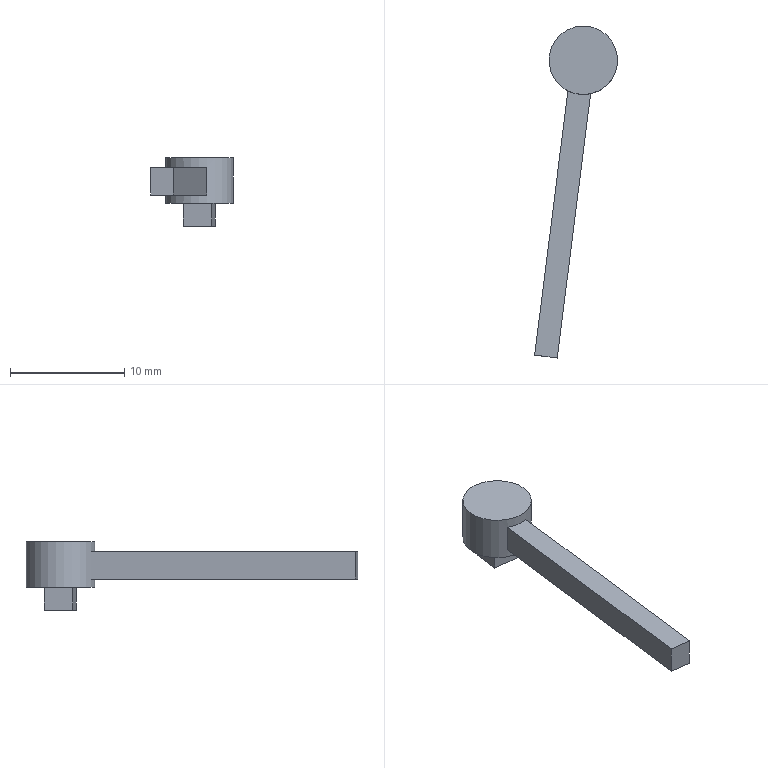Component | NX | HANDLE | 1 solid | 13 faces | box 7.27 x 29.03 x 6 mm | volume 237 mm3 | plane 12 | cylinder 1 | commonest cylinder face diameters 6 x1
STEP:
#1=CARTESIAN_POINT('',(0.,0.,0.));
#2=DIRECTION('',(0.,0.,1.));
#3=DIRECTION('',(1.,0.,0.));
#4=AXIS2_PLACEMENT_3D('',#1,#2,#3);
#5=CARTESIAN_POINT('',(33.486,50.648,24.212));
#6=VERTEX_POINT('',#5);
#7=CARTESIAN_POINT('',(30.51,51.025,24.212));
#8=DIRECTION('',(0.,0.,1.));
#9=DIRECTION('',(0.9921,-0.1255,0.));
#10=AXIS2_PLACEMENT_3D('',#7,#8,#9);
#11=CIRCLE('',#10,3.);
#12=CARTESIAN_POINT('',(30.51,51.025,24.212));
#13=DIRECTION('',(0.,0.,1.));
#14=DIRECTION('',(0.9921,-0.1255,0.));
#15=AXIS2_PLACEMENT_3D('',#12,#13,#14);
#16=CYLINDRICAL_SURFACE('',#15,3.);
#17=CARTESIAN_POINT('',(0.,0.));
#18=DIRECTION('',(1.,0.));
#19=VECTOR('',#18,1.);
#20=LINE('',#17,#19);
#21=(GEOMETRIC_REPRESENTATION_CONTEXT(2)PARAMETRIC_REPRESENTATION_CONTEXT()REPRESENTATION_CONTEXT('',''));
#22=DEFINITIONAL_REPRESENTATION('',(#20),#21);
#23=PCURVE('',#16,#22);
#24=CARTESIAN_POINT('',(30.51,51.025,24.212));
#25=DIRECTION('',(0.,0.,1.));
#26=DIRECTION('',(0.9921,-0.1255,0.));
#27=AXIS2_PLACEMENT_3D('',#24,#25,#26);
#28=PLANE('',#27);
#29=CARTESIAN_POINT('',(0.,0.));
#30=DIRECTION('',(1.,0.));
#31=AXIS2_PLACEMENT_2D('',#29,#30);
#32=CIRCLE('',#31,3.);
#33=(GEOMETRIC_REPRESENTATION_CONTEXT(2)PARAMETRIC_REPRESENTATION_CONTEXT()REPRESENTATION_CONTEXT('',''));
#34=DEFINITIONAL_REPRESENTATION('',(#32),#33);
#35=PCURVE('',#28,#34);
#36=SURFACE_CURVE('',#11,(#23,#35),.PCURVE_S1.);
#37=EDGE_CURVE('',#6,#6,#36,.T.);
#38=ORIENTED_EDGE('',*,*,#37,.T.);
#39=CARTESIAN_POINT('',(33.486,50.648,28.212));
#40=VERTEX_POINT('',#39);
#41=CARTESIAN_POINT('',(33.486,50.648,24.212));
#42=CARTESIAN_POINT('',(33.486,50.648,28.212));
#43=B_SPLINE_CURVE_WITH_KNOTS('',1,(#41,#42),.UNSPECIFIED.,.F.,.F.,(2,2),(0.,4.),.PIECEWISE_BEZIER_KNOTS.);
#44=CARTESIAN_POINT('',(6.283,0.));
#45=DIRECTION('',(0.,1.));
#46=VECTOR('',#45,1.);
#47=LINE('',#44,#46);
#48=(GEOMETRIC_REPRESENTATION_CONTEXT(2)PARAMETRIC_REPRESENTATION_CONTEXT()REPRESENTATION_CONTEXT('',''));
#49=DEFINITIONAL_REPRESENTATION('',(#47),#48);
#50=PCURVE('',#16,#49);
#51=CARTESIAN_POINT('',(0.,0.));
#52=DIRECTION('',(0.,1.));
#53=VECTOR('',#52,1.);
#54=LINE('',#51,#53);
#55=(GEOMETRIC_REPRESENTATION_CONTEXT(2)PARAMETRIC_REPRESENTATION_CONTEXT()REPRESENTATION_CONTEXT('',''));
#56=DEFINITIONAL_REPRESENTATION('',(#54),#55);
#57=PCURVE('',#16,#56);
#58=SEAM_CURVE('',#43,(#50,#57),.PCURVE_S1.);
#59=EDGE_CURVE('',#6,#40,#58,.T.);
#60=ORIENTED_EDGE('',*,*,#59,.T.);
#61=CARTESIAN_POINT('',(30.51,51.025,28.212));
#62=DIRECTION('',(0.,0.,1.));
#63=DIRECTION('',(0.9921,-0.1255,0.));
#64=AXIS2_PLACEMENT_3D('',#61,#62,#63);
#65=CIRCLE('',#64,3.);
#66=CARTESIAN_POINT('',(0.,4.));
#67=DIRECTION('',(1.,0.));
#68=VECTOR('',#67,1.);
#69=LINE('',#66,#68);
#70=(GEOMETRIC_REPRESENTATION_CONTEXT(2)PARAMETRIC_REPRESENTATION_CONTEXT()REPRESENTATION_CONTEXT('',''));
#71=DEFINITIONAL_REPRESENTATION('',(#69),#70);
#72=PCURVE('',#16,#71);
#73=CARTESIAN_POINT('',(30.51,51.025,28.212));
#74=DIRECTION('',(0.,0.,1.));
#75=DIRECTION('',(0.9921,-0.1255,0.));
#76=AXIS2_PLACEMENT_3D('',#73,#74,#75);
#77=PLANE('',#76);
#78=CARTESIAN_POINT('',(0.,0.));
#79=DIRECTION('',(1.,0.));
#80=AXIS2_PLACEMENT_2D('',#78,#79);
#81=CIRCLE('',#80,3.);
#82=(GEOMETRIC_REPRESENTATION_CONTEXT(2)PARAMETRIC_REPRESENTATION_CONTEXT()REPRESENTATION_CONTEXT('',''));
#83=DEFINITIONAL_REPRESENTATION('',(#81),#82);
#84=PCURVE('',#77,#83);
#85=SURFACE_CURVE('',#65,(#72,#84),.PCURVE_S1.);
#86=EDGE_CURVE('',#40,#40,#85,.T.);
#87=ORIENTED_EDGE('',*,*,#86,.F.);
#88=ORIENTED_EDGE('',*,*,#59,.F.);
#89=EDGE_LOOP('',(#38,#60,#87,#88));
#90=FACE_BOUND('',#89,.T.);
#91=CARTESIAN_POINT('',(29.163,48.344,24.948));
#92=VERTEX_POINT('',#91);
#93=CARTESIAN_POINT('',(31.147,48.093,24.948));
#94=VERTEX_POINT('',#93);
#95=CARTESIAN_POINT('',(30.51,51.025,24.948));
#96=DIRECTION('',(0.,0.,1.));
#97=DIRECTION('',(-0.9921,0.1255,0.));
#98=AXIS2_PLACEMENT_3D('',#95,#96,#97);
#99=CIRCLE('',#98,3.);
#100=CARTESIAN_POINT('',(3.142,0.7363));
#101=DIRECTION('',(1.,0.));
#102=VECTOR('',#101,1.);
#103=LINE('',#100,#102);
#104=(GEOMETRIC_REPRESENTATION_CONTEXT(2)PARAMETRIC_REPRESENTATION_CONTEXT()REPRESENTATION_CONTEXT('',''));
#105=DEFINITIONAL_REPRESENTATION('',(#103),#104);
#106=PCURVE('',#16,#105);
#107=CARTESIAN_POINT('',(26.242,25.242,24.948));
#108=DIRECTION('',(0.,0.,-1.));
#109=DIRECTION('',(-0.9921,0.1255,0.));
#110=AXIS2_PLACEMENT_3D('',#107,#108,#109);
#111=PLANE('',#110);
#112=CARTESIAN_POINT('',(2.,26.115));
#113=CARTESIAN_POINT('',(2.,20.919));
#114=CARTESIAN_POINT('',(-2.5,23.517));
#115=CARTESIAN_POINT('',(-7.,26.115));
#116=CARTESIAN_POINT('',(-2.5,28.713));
#117=CARTESIAN_POINT('',(2.,31.311));
#118=CARTESIAN_POINT('',(2.,26.115));
#119=(BOUNDED_CURVE()B_SPLINE_CURVE(2,(#112,#113,#114,#115,#116,#117,#118),.UNSPECIFIED.,.T.,.F.)B_SPLINE_CURVE_WITH_KNOTS((1,2,2,2,2,1),(-2.094,0.,2.094,4.189,6.283,8.378),.UNSPECIFIED.)CURVE()GEOMETRIC_REPRESENTATION_ITEM()RATIONAL_B_SPLINE_CURVE((1.,0.5,1.,0.5,1.,0.5,1.))REPRESENTATION_ITEM(''));
#120=(GEOMETRIC_REPRESENTATION_CONTEXT(2)PARAMETRIC_REPRESENTATION_CONTEXT()REPRESENTATION_CONTEXT('',''));
#121=DEFINITIONAL_REPRESENTATION('',(#119),#120);
#122=PCURVE('',#111,#121);
#123=SURFACE_CURVE('',#99,(#106,#122),.PCURVE_S1.);
#124=EDGE_CURVE('',#92,#94,#123,.T.);
#125=ORIENTED_EDGE('',*,*,#124,.F.);
#126=CARTESIAN_POINT('',(29.163,48.344,27.342));
#127=VERTEX_POINT('',#126);
#128=CARTESIAN_POINT('',(29.163,48.344,24.212));
#129=DIRECTION('',(0.,0.,1.));
#130=VECTOR('',#129,1.);
#131=LINE('',#128,#130);
#132=CARTESIAN_POINT('',(4.373,0.));
#133=DIRECTION('',(0.,1.));
#134=VECTOR('',#133,1.);
#135=LINE('',#132,#134);
#136=(GEOMETRIC_REPRESENTATION_CONTEXT(2)PARAMETRIC_REPRESENTATION_CONTEXT()REPRESENTATION_CONTEXT('',''));
#137=DEFINITIONAL_REPRESENTATION('',(#135),#136);
#138=PCURVE('',#16,#137);
#139=CARTESIAN_POINT('',(29.518,51.15,24.212));
#140=DIRECTION('',(0.9921,-0.1255,0.));
#141=DIRECTION('',(0.,0.,-1.));
#142=AXIS2_PLACEMENT_3D('',#139,#140,#141);
#143=PLANE('',#142);
#144=CARTESIAN_POINT('',(0.,-2.828));
#145=DIRECTION('',(-1.,0.));
#146=VECTOR('',#145,1.);
#147=LINE('',#144,#146);
#148=(GEOMETRIC_REPRESENTATION_CONTEXT(2)PARAMETRIC_REPRESENTATION_CONTEXT()REPRESENTATION_CONTEXT('',''));
#149=DEFINITIONAL_REPRESENTATION('',(#147),#148);
#150=PCURVE('',#143,#149);
#151=SURFACE_CURVE('',#131,(#138,#150),.PCURVE_S1.);
#152=EDGE_CURVE('',#92,#127,#151,.T.);
#153=ORIENTED_EDGE('',*,*,#152,.T.);
#154=CARTESIAN_POINT('',(31.147,48.093,27.342));
#155=VERTEX_POINT('',#154);
#156=CARTESIAN_POINT('',(30.51,51.025,27.342));
#157=DIRECTION('',(0.,0.,-1.));
#158=DIRECTION('',(-0.1255,-0.9921,-0.));
#159=AXIS2_PLACEMENT_3D('',#156,#157,#158);
#160=CIRCLE('',#159,3.);
#161=CARTESIAN_POINT('',(10.996,3.13));
#162=DIRECTION('',(-1.,0.));
#163=VECTOR('',#162,1.);
#164=LINE('',#161,#163);
#165=(GEOMETRIC_REPRESENTATION_CONTEXT(2)PARAMETRIC_REPRESENTATION_CONTEXT()REPRESENTATION_CONTEXT('',''));
#166=DEFINITIONAL_REPRESENTATION('',(#164),#165);
#167=PCURVE('',#16,#166);
#168=CARTESIAN_POINT('',(29.417,50.356,27.342));
#169=DIRECTION('',(-0.,-0.,1.));
#170=DIRECTION('',(-0.1255,-0.9921,-0.));
#171=AXIS2_PLACEMENT_3D('',#168,#169,#170);
#172=PLANE('',#171);
#173=CARTESIAN_POINT('',(2.2,1.));
#174=CARTESIAN_POINT('',(2.2,-4.196));
#175=CARTESIAN_POINT('',(-2.3,-1.598));
#176=CARTESIAN_POINT('',(-6.8,1.));
#177=CARTESIAN_POINT('',(-2.3,3.598));
#178=CARTESIAN_POINT('',(2.2,6.196));
#179=CARTESIAN_POINT('',(2.2,1.));
#180=(BOUNDED_CURVE()B_SPLINE_CURVE(2,(#173,#174,#175,#176,#177,#178,#179),.UNSPECIFIED.,.T.,.F.)B_SPLINE_CURVE_WITH_KNOTS((1,2,2,2,2,1),(-2.094,0.,2.094,4.189,6.283,8.378),.UNSPECIFIED.)CURVE()GEOMETRIC_REPRESENTATION_ITEM()RATIONAL_B_SPLINE_CURVE((1.,0.5,1.,0.5,1.,0.5,1.))REPRESENTATION_ITEM(''));
#181=(GEOMETRIC_REPRESENTATION_CONTEXT(2)PARAMETRIC_REPRESENTATION_CONTEXT()REPRESENTATION_CONTEXT('',''));
#182=DEFINITIONAL_REPRESENTATION('',(#180),#181);
#183=PCURVE('',#172,#182);
#184=SURFACE_CURVE('',#160,(#167,#183),.PCURVE_S1.);
#185=EDGE_CURVE('',#155,#127,#184,.T.);
#186=ORIENTED_EDGE('',*,*,#185,.F.);
#187=CARTESIAN_POINT('',(31.147,48.093,24.212));
#188=DIRECTION('',(0.,0.,1.));
#189=VECTOR('',#188,1.);
#190=LINE('',#187,#189);
#191=CARTESIAN_POINT('',(5.052,0.));
#192=DIRECTION('',(0.,1.));
#193=VECTOR('',#192,1.);
#194=LINE('',#191,#193);
#195=(GEOMETRIC_REPRESENTATION_CONTEXT(2)PARAMETRIC_REPRESENTATION_CONTEXT()REPRESENTATION_CONTEXT('',''));
#196=DEFINITIONAL_REPRESENTATION('',(#194),#195);
#197=PCURVE('',#16,#196);
#198=CARTESIAN_POINT('',(31.502,50.899,24.212));
#199=DIRECTION('',(0.9921,-0.1255,0.));
#200=DIRECTION('',(0.,0.,-1.));
#201=AXIS2_PLACEMENT_3D('',#198,#199,#200);
#202=PLANE('',#201);
#203=CARTESIAN_POINT('',(0.,-2.828));
#204=DIRECTION('',(-1.,0.));
#205=VECTOR('',#204,1.);
#206=LINE('',#203,#205);
#207=(GEOMETRIC_REPRESENTATION_CONTEXT(2)PARAMETRIC_REPRESENTATION_CONTEXT()REPRESENTATION_CONTEXT('',''));
#208=DEFINITIONAL_REPRESENTATION('',(#206),#207);
#209=PCURVE('',#202,#208);
#210=SURFACE_CURVE('',#190,(#197,#209),.PCURVE_S1.);
#211=EDGE_CURVE('',#94,#155,#210,.T.);
#212=ORIENTED_EDGE('',*,*,#211,.F.);
#213=EDGE_LOOP('',(#125,#153,#186,#212));
#214=FACE_BOUND('',#213,.T.);
#215=ADVANCED_FACE('',(#90,#214),#16,.T.);
#216=ORIENTED_EDGE('',*,*,#37,.F.);
#217=EDGE_LOOP('',(#216));
#218=FACE_BOUND('',#217,.T.);
#219=CARTESIAN_POINT('',(29.113,49.941,24.212));
#220=VERTEX_POINT('',#219);
#221=CARTESIAN_POINT('',(29.427,52.422,24.212));
#222=VERTEX_POINT('',#221);
#223=CARTESIAN_POINT('',(29.113,49.941,24.212));
#224=DIRECTION('',(0.1255,0.9921,0.));
#225=VECTOR('',#224,1.);
#226=LINE('',#223,#225);
#227=CARTESIAN_POINT('',(-1.25,-1.25));
#228=DIRECTION('',(0.,1.));
#229=VECTOR('',#228,1.);
#230=LINE('',#227,#229);
#231=(GEOMETRIC_REPRESENTATION_CONTEXT(2)PARAMETRIC_REPRESENTATION_CONTEXT()REPRESENTATION_CONTEXT('',''));
#232=DEFINITIONAL_REPRESENTATION('',(#230),#231);
#233=PCURVE('',#28,#232);
#234=CARTESIAN_POINT('',(29.427,52.422,22.212));
#235=DIRECTION('',(-0.9921,0.1255,0.));
#236=DIRECTION('',(0.,0.,1.));
#237=AXIS2_PLACEMENT_3D('',#234,#235,#236);
#238=PLANE('',#237);
#239=CARTESIAN_POINT('',(2.,-2.5));
#240=DIRECTION('',(0.,1.));
#241=VECTOR('',#240,1.);
#242=LINE('',#239,#241);
#243=(GEOMETRIC_REPRESENTATION_CONTEXT(2)PARAMETRIC_REPRESENTATION_CONTEXT()REPRESENTATION_CONTEXT('',''));
#244=DEFINITIONAL_REPRESENTATION('',(#242),#243);
#245=PCURVE('',#238,#244);
#246=SURFACE_CURVE('',#226,(#233,#245),.PCURVE_S1.);
#247=EDGE_CURVE('',#220,#222,#246,.T.);
#248=ORIENTED_EDGE('',*,*,#247,.F.);
#249=CARTESIAN_POINT('',(31.593,49.628,24.212));
#250=VERTEX_POINT('',#249);
#251=CARTESIAN_POINT('',(31.593,49.628,24.212));
#252=DIRECTION('',(-0.9921,0.1255,0.));
#253=VECTOR('',#252,1.);
#254=LINE('',#251,#253);
#255=CARTESIAN_POINT('',(1.25,-1.25));
#256=DIRECTION('',(-1.,0.));
#257=VECTOR('',#256,1.);
#258=LINE('',#255,#257);
#259=(GEOMETRIC_REPRESENTATION_CONTEXT(2)PARAMETRIC_REPRESENTATION_CONTEXT()REPRESENTATION_CONTEXT('',''));
#260=DEFINITIONAL_REPRESENTATION('',(#258),#259);
#261=PCURVE('',#28,#260);
#262=CARTESIAN_POINT('',(29.113,49.941,22.212));
#263=DIRECTION('',(-0.1255,-0.9921,0.));
#264=DIRECTION('',(0.9921,-0.1255,0.));
#265=AXIS2_PLACEMENT_3D('',#262,#263,#264);
#266=PLANE('',#265);
#267=CARTESIAN_POINT('',(2.5,2.));
#268=DIRECTION('',(-1.,0.));
#269=VECTOR('',#268,1.);
#270=LINE('',#267,#269);
#271=(GEOMETRIC_REPRESENTATION_CONTEXT(2)PARAMETRIC_REPRESENTATION_CONTEXT()REPRESENTATION_CONTEXT('',''));
#272=DEFINITIONAL_REPRESENTATION('',(#270),#271);
#273=PCURVE('',#266,#272);
#274=SURFACE_CURVE('',#254,(#261,#273),.PCURVE_S1.);
#275=EDGE_CURVE('',#250,#220,#274,.T.);
#276=ORIENTED_EDGE('',*,*,#275,.F.);
#277=CARTESIAN_POINT('',(31.907,52.108,24.212));
#278=VERTEX_POINT('',#277);
#279=CARTESIAN_POINT('',(31.907,52.108,24.212));
#280=DIRECTION('',(-0.1255,-0.9921,0.));
#281=VECTOR('',#280,1.);
#282=LINE('',#279,#281);
#283=CARTESIAN_POINT('',(1.25,1.25));
#284=DIRECTION('',(0.,-1.));
#285=VECTOR('',#284,1.);
#286=LINE('',#283,#285);
#287=(GEOMETRIC_REPRESENTATION_CONTEXT(2)PARAMETRIC_REPRESENTATION_CONTEXT()REPRESENTATION_CONTEXT('',''));
#288=DEFINITIONAL_REPRESENTATION('',(#286),#287);
#289=PCURVE('',#28,#288);
#290=CARTESIAN_POINT('',(31.593,49.628,22.212));
#291=DIRECTION('',(0.9921,-0.1255,0.));
#292=DIRECTION('',(0.1255,0.9921,0.));
#293=AXIS2_PLACEMENT_3D('',#290,#291,#292);
#294=PLANE('',#293);
#295=CARTESIAN_POINT('',(2.5,2.));
#296=DIRECTION('',(-1.,0.));
#297=VECTOR('',#296,1.);
#298=LINE('',#295,#297);
#299=(GEOMETRIC_REPRESENTATION_CONTEXT(2)PARAMETRIC_REPRESENTATION_CONTEXT()REPRESENTATION_CONTEXT('',''));
#300=DEFINITIONAL_REPRESENTATION('',(#298),#299);
#301=PCURVE('',#294,#300);
#302=SURFACE_CURVE('',#282,(#289,#301),.PCURVE_S1.);
#303=EDGE_CURVE('',#278,#250,#302,.T.);
#304=ORIENTED_EDGE('',*,*,#303,.F.);
#305=CARTESIAN_POINT('',(29.427,52.422,24.212));
#306=DIRECTION('',(0.9921,-0.1255,0.));
#307=VECTOR('',#306,1.);
#308=LINE('',#305,#307);
#309=CARTESIAN_POINT('',(-1.25,1.25));
#310=DIRECTION('',(1.,0.));
#311=VECTOR('',#310,1.);
#312=LINE('',#309,#311);
#313=(GEOMETRIC_REPRESENTATION_CONTEXT(2)PARAMETRIC_REPRESENTATION_CONTEXT()REPRESENTATION_CONTEXT('',''));
#314=DEFINITIONAL_REPRESENTATION('',(#312),#313);
#315=PCURVE('',#28,#314);
#316=CARTESIAN_POINT('',(31.907,52.108,22.212));
#317=DIRECTION('',(0.1255,0.9921,0.));
#318=DIRECTION('',(-0.9921,0.1255,0.));
#319=AXIS2_PLACEMENT_3D('',#316,#317,#318);
#320=PLANE('',#319);
#321=CARTESIAN_POINT('',(2.5,2.));
#322=DIRECTION('',(-1.,0.));
#323=VECTOR('',#322,1.);
#324=LINE('',#321,#323);
#325=(GEOMETRIC_REPRESENTATION_CONTEXT(2)PARAMETRIC_REPRESENTATION_CONTEXT()REPRESENTATION_CONTEXT('',''));
#326=DEFINITIONAL_REPRESENTATION('',(#324),#325);
#327=PCURVE('',#320,#326);
#328=SURFACE_CURVE('',#308,(#315,#327),.PCURVE_S1.);
#329=EDGE_CURVE('',#222,#278,#328,.T.);
#330=ORIENTED_EDGE('',*,*,#329,.F.);
#331=EDGE_LOOP('',(#248,#276,#304,#330));
#332=FACE_BOUND('',#331,.T.);
#333=ADVANCED_FACE('',(#218,#332),#28,.F.);
#334=ORIENTED_EDGE('',*,*,#86,.T.);
#335=EDGE_LOOP('',(#334));
#336=FACE_BOUND('',#335,.T.);
#337=ADVANCED_FACE('',(#336),#77,.T.);
#338=CARTESIAN_POINT('',(29.427,52.422,22.212));
#339=VERTEX_POINT('',#338);
#340=CARTESIAN_POINT('',(29.113,49.941,22.212));
#341=VERTEX_POINT('',#340);
#342=CARTESIAN_POINT('',(29.427,52.422,22.212));
#343=DIRECTION('',(-0.1255,-0.9921,0.));
#344=VECTOR('',#343,1.);
#345=LINE('',#342,#344);
#346=CARTESIAN_POINT('',(30.51,51.025,22.212));
#347=DIRECTION('',(0.,0.,1.));
#348=DIRECTION('',(0.9921,-0.1255,0.));
#349=AXIS2_PLACEMENT_3D('',#346,#347,#348);
#350=PLANE('',#349);
#351=CARTESIAN_POINT('',(-1.25,1.25));
#352=DIRECTION('',(0.,-1.));
#353=VECTOR('',#352,1.);
#354=LINE('',#351,#353);
#355=(GEOMETRIC_REPRESENTATION_CONTEXT(2)PARAMETRIC_REPRESENTATION_CONTEXT()REPRESENTATION_CONTEXT('',''));
#356=DEFINITIONAL_REPRESENTATION('',(#354),#355);
#357=PCURVE('',#350,#356);
#358=CARTESIAN_POINT('',(0.,0.));
#359=DIRECTION('',(0.,-1.));
#360=VECTOR('',#359,1.);
#361=LINE('',#358,#360);
#362=(GEOMETRIC_REPRESENTATION_CONTEXT(2)PARAMETRIC_REPRESENTATION_CONTEXT()REPRESENTATION_CONTEXT('',''));
#363=DEFINITIONAL_REPRESENTATION('',(#361),#362);
#364=PCURVE('',#238,#363);
#365=SURFACE_CURVE('',#345,(#357,#364),.PCURVE_S1.);
#366=EDGE_CURVE('',#339,#341,#365,.T.);
#367=ORIENTED_EDGE('',*,*,#366,.F.);
#368=CARTESIAN_POINT('',(31.907,52.108,22.212));
#369=VERTEX_POINT('',#368);
#370=CARTESIAN_POINT('',(31.907,52.108,22.212));
#371=DIRECTION('',(-0.9921,0.1255,0.));
#372=VECTOR('',#371,1.);
#373=LINE('',#370,#372);
#374=CARTESIAN_POINT('',(1.25,1.25));
#375=DIRECTION('',(-1.,0.));
#376=VECTOR('',#375,1.);
#377=LINE('',#374,#376);
#378=(GEOMETRIC_REPRESENTATION_CONTEXT(2)PARAMETRIC_REPRESENTATION_CONTEXT()REPRESENTATION_CONTEXT('',''));
#379=DEFINITIONAL_REPRESENTATION('',(#377),#378);
#380=PCURVE('',#350,#379);
#381=CARTESIAN_POINT('',(0.,0.));
#382=DIRECTION('',(1.,0.));
#383=VECTOR('',#382,1.);
#384=LINE('',#381,#383);
#385=(GEOMETRIC_REPRESENTATION_CONTEXT(2)PARAMETRIC_REPRESENTATION_CONTEXT()REPRESENTATION_CONTEXT('',''));
#386=DEFINITIONAL_REPRESENTATION('',(#384),#385);
#387=PCURVE('',#320,#386);
#388=SURFACE_CURVE('',#373,(#380,#387),.PCURVE_S1.);
#389=EDGE_CURVE('',#369,#339,#388,.T.);
#390=ORIENTED_EDGE('',*,*,#389,.F.);
#391=CARTESIAN_POINT('',(31.593,49.628,22.212));
#392=VERTEX_POINT('',#391);
#393=CARTESIAN_POINT('',(31.593,49.628,22.212));
#394=DIRECTION('',(0.1255,0.9921,0.));
#395=VECTOR('',#394,1.);
#396=LINE('',#393,#395);
#397=CARTESIAN_POINT('',(1.25,-1.25));
#398=DIRECTION('',(0.,1.));
#399=VECTOR('',#398,1.);
#400=LINE('',#397,#399);
#401=(GEOMETRIC_REPRESENTATION_CONTEXT(2)PARAMETRIC_REPRESENTATION_CONTEXT()REPRESENTATION_CONTEXT('',''));
#402=DEFINITIONAL_REPRESENTATION('',(#400),#401);
#403=PCURVE('',#350,#402);
#404=CARTESIAN_POINT('',(0.,0.));
#405=DIRECTION('',(1.,0.));
#406=VECTOR('',#405,1.);
#407=LINE('',#404,#406);
#408=(GEOMETRIC_REPRESENTATION_CONTEXT(2)PARAMETRIC_REPRESENTATION_CONTEXT()REPRESENTATION_CONTEXT('',''));
#409=DEFINITIONAL_REPRESENTATION('',(#407),#408);
#410=PCURVE('',#294,#409);
#411=SURFACE_CURVE('',#396,(#403,#410),.PCURVE_S1.);
#412=EDGE_CURVE('',#392,#369,#411,.T.);
#413=ORIENTED_EDGE('',*,*,#412,.F.);
#414=CARTESIAN_POINT('',(29.113,49.941,22.212));
#415=DIRECTION('',(0.9921,-0.1255,0.));
#416=VECTOR('',#415,1.);
#417=LINE('',#414,#416);
#418=CARTESIAN_POINT('',(-1.25,-1.25));
#419=DIRECTION('',(1.,0.));
#420=VECTOR('',#419,1.);
#421=LINE('',#418,#420);
#422=(GEOMETRIC_REPRESENTATION_CONTEXT(2)PARAMETRIC_REPRESENTATION_CONTEXT()REPRESENTATION_CONTEXT('',''));
#423=DEFINITIONAL_REPRESENTATION('',(#421),#422);
#424=PCURVE('',#350,#423);
#425=CARTESIAN_POINT('',(0.,0.));
#426=DIRECTION('',(1.,0.));
#427=VECTOR('',#426,1.);
#428=LINE('',#425,#427);
#429=(GEOMETRIC_REPRESENTATION_CONTEXT(2)PARAMETRIC_REPRESENTATION_CONTEXT()REPRESENTATION_CONTEXT('',''));
#430=DEFINITIONAL_REPRESENTATION('',(#428),#429);
#431=PCURVE('',#266,#430);
#432=SURFACE_CURVE('',#417,(#424,#431),.PCURVE_S1.);
#433=EDGE_CURVE('',#341,#392,#432,.T.);
#434=ORIENTED_EDGE('',*,*,#433,.F.);
#435=EDGE_LOOP('',(#367,#390,#413,#434));
#436=FACE_BOUND('',#435,.T.);
#437=ADVANCED_FACE('',(#436),#350,.F.);
#438=ORIENTED_EDGE('',*,*,#329,.T.);
#439=CARTESIAN_POINT('',(31.907,52.108,22.212));
#440=DIRECTION('',(0.,0.,1.));
#441=VECTOR('',#440,1.);
#442=LINE('',#439,#441);
#443=CARTESIAN_POINT('',(0.,0.));
#444=DIRECTION('',(0.,1.));
#445=VECTOR('',#444,1.);
#446=LINE('',#443,#445);
#447=(GEOMETRIC_REPRESENTATION_CONTEXT(2)PARAMETRIC_REPRESENTATION_CONTEXT()REPRESENTATION_CONTEXT('',''));
#448=DEFINITIONAL_REPRESENTATION('',(#446),#447);
#449=PCURVE('',#320,#448);
#450=CARTESIAN_POINT('',(2.5,0.));
#451=DIRECTION('',(0.,1.));
#452=VECTOR('',#451,1.);
#453=LINE('',#450,#452);
#454=(GEOMETRIC_REPRESENTATION_CONTEXT(2)PARAMETRIC_REPRESENTATION_CONTEXT()REPRESENTATION_CONTEXT('',''));
#455=DEFINITIONAL_REPRESENTATION('',(#453),#454);
#456=PCURVE('',#294,#455);
#457=SURFACE_CURVE('',#442,(#449,#456),.PCURVE_S1.);
#458=EDGE_CURVE('',#369,#278,#457,.T.);
#459=ORIENTED_EDGE('',*,*,#458,.F.);
#460=ORIENTED_EDGE('',*,*,#389,.T.);
#461=CARTESIAN_POINT('',(29.427,52.422,22.212));
#462=DIRECTION('',(0.,0.,1.));
#463=VECTOR('',#462,1.);
#464=LINE('',#461,#463);
#465=CARTESIAN_POINT('',(2.5,0.));
#466=DIRECTION('',(0.,1.));
#467=VECTOR('',#466,1.);
#468=LINE('',#465,#467);
#469=(GEOMETRIC_REPRESENTATION_CONTEXT(2)PARAMETRIC_REPRESENTATION_CONTEXT()REPRESENTATION_CONTEXT('',''));
#470=DEFINITIONAL_REPRESENTATION('',(#468),#469);
#471=PCURVE('',#320,#470);
#472=CARTESIAN_POINT('',(0.,0.));
#473=DIRECTION('',(1.,0.));
#474=VECTOR('',#473,1.);
#475=LINE('',#472,#474);
#476=(GEOMETRIC_REPRESENTATION_CONTEXT(2)PARAMETRIC_REPRESENTATION_CONTEXT()REPRESENTATION_CONTEXT('',''));
#477=DEFINITIONAL_REPRESENTATION('',(#475),#476);
#478=PCURVE('',#238,#477);
#479=SURFACE_CURVE('',#464,(#471,#478),.PCURVE_S1.);
#480=EDGE_CURVE('',#339,#222,#479,.T.);
#481=ORIENTED_EDGE('',*,*,#480,.T.);
#482=EDGE_LOOP('',(#438,#459,#460,#481));
#483=FACE_BOUND('',#482,.T.);
#484=ADVANCED_FACE('',(#483),#320,.T.);
#485=ORIENTED_EDGE('',*,*,#303,.T.);
#486=CARTESIAN_POINT('',(31.593,49.628,22.212));
#487=DIRECTION('',(0.,0.,1.));
#488=VECTOR('',#487,1.);
#489=LINE('',#486,#488);
#490=CARTESIAN_POINT('',(0.,0.));
#491=DIRECTION('',(0.,1.));
#492=VECTOR('',#491,1.);
#493=LINE('',#490,#492);
#494=(GEOMETRIC_REPRESENTATION_CONTEXT(2)PARAMETRIC_REPRESENTATION_CONTEXT()REPRESENTATION_CONTEXT('',''));
#495=DEFINITIONAL_REPRESENTATION('',(#493),#494);
#496=PCURVE('',#294,#495);
#497=CARTESIAN_POINT('',(2.5,0.));
#498=DIRECTION('',(0.,1.));
#499=VECTOR('',#498,1.);
#500=LINE('',#497,#499);
#501=(GEOMETRIC_REPRESENTATION_CONTEXT(2)PARAMETRIC_REPRESENTATION_CONTEXT()REPRESENTATION_CONTEXT('',''));
#502=DEFINITIONAL_REPRESENTATION('',(#500),#501);
#503=PCURVE('',#266,#502);
#504=SURFACE_CURVE('',#489,(#496,#503),.PCURVE_S1.);
#505=EDGE_CURVE('',#392,#250,#504,.T.);
#506=ORIENTED_EDGE('',*,*,#505,.F.);
#507=ORIENTED_EDGE('',*,*,#412,.T.);
#508=ORIENTED_EDGE('',*,*,#458,.T.);
#509=EDGE_LOOP('',(#485,#506,#507,#508));
#510=FACE_BOUND('',#509,.T.);
#511=ADVANCED_FACE('',(#510),#294,.T.);
#512=ORIENTED_EDGE('',*,*,#275,.T.);
#513=CARTESIAN_POINT('',(29.113,49.941,22.212));
#514=DIRECTION('',(0.,0.,1.));
#515=VECTOR('',#514,1.);
#516=LINE('',#513,#515);
#517=CARTESIAN_POINT('',(0.,0.));
#518=DIRECTION('',(0.,1.));
#519=VECTOR('',#518,1.);
#520=LINE('',#517,#519);
#521=(GEOMETRIC_REPRESENTATION_CONTEXT(2)PARAMETRIC_REPRESENTATION_CONTEXT()REPRESENTATION_CONTEXT('',''));
#522=DEFINITIONAL_REPRESENTATION('',(#520),#521);
#523=PCURVE('',#266,#522);
#524=CARTESIAN_POINT('',(0.,-2.5));
#525=DIRECTION('',(1.,0.));
#526=VECTOR('',#525,1.);
#527=LINE('',#524,#526);
#528=(GEOMETRIC_REPRESENTATION_CONTEXT(2)PARAMETRIC_REPRESENTATION_CONTEXT()REPRESENTATION_CONTEXT('',''));
#529=DEFINITIONAL_REPRESENTATION('',(#527),#528);
#530=PCURVE('',#238,#529);
#531=SURFACE_CURVE('',#516,(#523,#530),.PCURVE_S1.);
#532=EDGE_CURVE('',#341,#220,#531,.T.);
#533=ORIENTED_EDGE('',*,*,#532,.F.);
#534=ORIENTED_EDGE('',*,*,#433,.T.);
#535=ORIENTED_EDGE('',*,*,#505,.T.);
#536=EDGE_LOOP('',(#512,#533,#534,#535));
#537=FACE_BOUND('',#536,.T.);
#538=ADVANCED_FACE('',(#537),#266,.T.);
#539=ORIENTED_EDGE('',*,*,#247,.T.);
#540=ORIENTED_EDGE('',*,*,#480,.F.);
#541=ORIENTED_EDGE('',*,*,#366,.T.);
#542=ORIENTED_EDGE('',*,*,#532,.T.);
#543=EDGE_LOOP('',(#539,#540,#541,#542));
#544=FACE_BOUND('',#543,.T.);
#545=ADVANCED_FACE('',(#544),#238,.T.);
#546=CARTESIAN_POINT('',(28.226,24.991,27.342));
#547=VERTEX_POINT('',#546);
#548=CARTESIAN_POINT('',(28.226,24.991,24.948));
#549=VERTEX_POINT('',#548);
#550=CARTESIAN_POINT('',(28.226,24.991,27.342));
#551=DIRECTION('',(0.,0.,-1.));
#552=VECTOR('',#551,1.);
#553=LINE('',#550,#552);
#554=CARTESIAN_POINT('',(26.242,25.242,27.342));
#555=DIRECTION('',(-0.1255,-0.9921,0.));
#556=DIRECTION('',(0.,0.,-1.));
#557=AXIS2_PLACEMENT_3D('',#554,#555,#556);
#558=PLANE('',#557);
#559=CARTESIAN_POINT('',(0.,2.));
#560=DIRECTION('',(1.,0.));
#561=VECTOR('',#560,1.);
#562=LINE('',#559,#561);
#563=(GEOMETRIC_REPRESENTATION_CONTEXT(2)PARAMETRIC_REPRESENTATION_CONTEXT()REPRESENTATION_CONTEXT('',''));
#564=DEFINITIONAL_REPRESENTATION('',(#562),#563);
#565=PCURVE('',#558,#564);
#566=CARTESIAN_POINT('',(-3.13,-26.115));
#567=DIRECTION('',(1.,0.));
#568=VECTOR('',#567,1.);
#569=LINE('',#566,#568);
#570=(GEOMETRIC_REPRESENTATION_CONTEXT(2)PARAMETRIC_REPRESENTATION_CONTEXT()REPRESENTATION_CONTEXT('',''));
#571=DEFINITIONAL_REPRESENTATION('',(#569),#570);
#572=PCURVE('',#202,#571);
#573=SURFACE_CURVE('',#553,(#565,#572),.PCURVE_S1.);
#574=EDGE_CURVE('',#547,#549,#573,.T.);
#575=ORIENTED_EDGE('',*,*,#574,.F.);
#576=CARTESIAN_POINT('',(26.242,25.242,27.342));
#577=VERTEX_POINT('',#576);
#578=CARTESIAN_POINT('',(26.242,25.242,27.342));
#579=DIRECTION('',(0.9921,-0.1255,0.));
#580=VECTOR('',#579,1.);
#581=LINE('',#578,#580);
#582=CARTESIAN_POINT('',(0.,0.));
#583=DIRECTION('',(0.,1.));
#584=VECTOR('',#583,1.);
#585=LINE('',#582,#584);
#586=(GEOMETRIC_REPRESENTATION_CONTEXT(2)PARAMETRIC_REPRESENTATION_CONTEXT()REPRESENTATION_CONTEXT('',''));
#587=DEFINITIONAL_REPRESENTATION('',(#585),#586);
#588=PCURVE('',#558,#587);
#589=CARTESIAN_POINT('',(25.315,0.));
#590=DIRECTION('',(0.,1.));
#591=VECTOR('',#590,1.);
#592=LINE('',#589,#591);
#593=(GEOMETRIC_REPRESENTATION_CONTEXT(2)PARAMETRIC_REPRESENTATION_CONTEXT()REPRESENTATION_CONTEXT('',''));
#594=DEFINITIONAL_REPRESENTATION('',(#592),#593);
#595=PCURVE('',#172,#594);
#596=SURFACE_CURVE('',#581,(#588,#595),.PCURVE_S1.);
#597=EDGE_CURVE('',#577,#547,#596,.T.);
#598=ORIENTED_EDGE('',*,*,#597,.F.);
#599=CARTESIAN_POINT('',(26.242,25.242,24.948));
#600=VERTEX_POINT('',#599);
#601=CARTESIAN_POINT('',(26.242,25.242,27.342));
#602=DIRECTION('',(0.,0.,-1.));
#603=VECTOR('',#602,1.);
#604=LINE('',#601,#603);
#605=CARTESIAN_POINT('',(0.,0.));
#606=DIRECTION('',(1.,0.));
#607=VECTOR('',#606,1.);
#608=LINE('',#605,#607);
#609=(GEOMETRIC_REPRESENTATION_CONTEXT(2)PARAMETRIC_REPRESENTATION_CONTEXT()REPRESENTATION_CONTEXT('',''));
#610=DEFINITIONAL_REPRESENTATION('',(#608),#609);
#611=PCURVE('',#558,#610);
#612=CARTESIAN_POINT('',(-3.13,-26.115));
#613=DIRECTION('',(1.,0.));
#614=VECTOR('',#613,1.);
#615=LINE('',#612,#614);
#616=(GEOMETRIC_REPRESENTATION_CONTEXT(2)PARAMETRIC_REPRESENTATION_CONTEXT()REPRESENTATION_CONTEXT('',''));
#617=DEFINITIONAL_REPRESENTATION('',(#615),#616);
#618=PCURVE('',#143,#617);
#619=SURFACE_CURVE('',#604,(#611,#618),.PCURVE_S1.);
#620=EDGE_CURVE('',#577,#600,#619,.T.);
#621=ORIENTED_EDGE('',*,*,#620,.T.);
#622=CARTESIAN_POINT('',(26.242,25.242,24.948));
#623=DIRECTION('',(0.9921,-0.1255,0.));
#624=VECTOR('',#623,1.);
#625=LINE('',#622,#624);
#626=CARTESIAN_POINT('',(2.394,0.));
#627=DIRECTION('',(0.,1.));
#628=VECTOR('',#627,1.);
#629=LINE('',#626,#628);
#630=(GEOMETRIC_REPRESENTATION_CONTEXT(2)PARAMETRIC_REPRESENTATION_CONTEXT()REPRESENTATION_CONTEXT('',''));
#631=DEFINITIONAL_REPRESENTATION('',(#629),#630);
#632=PCURVE('',#558,#631);
#633=CARTESIAN_POINT('',(0.,0.));
#634=DIRECTION('',(-1.,0.));
#635=VECTOR('',#634,1.);
#636=LINE('',#633,#635);
#637=(GEOMETRIC_REPRESENTATION_CONTEXT(2)PARAMETRIC_REPRESENTATION_CONTEXT()REPRESENTATION_CONTEXT('',''));
#638=DEFINITIONAL_REPRESENTATION('',(#636),#637);
#639=PCURVE('',#111,#638);
#640=SURFACE_CURVE('',#625,(#632,#639),.PCURVE_S1.);
#641=EDGE_CURVE('',#600,#549,#640,.T.);
#642=ORIENTED_EDGE('',*,*,#641,.T.);
#643=EDGE_LOOP('',(#575,#598,#621,#642));
#644=FACE_BOUND('',#643,.T.);
#645=ADVANCED_FACE('',(#644),#558,.T.);
#646=CARTESIAN_POINT('',(26.242,25.242,24.948));
#647=DIRECTION('',(0.1255,0.9921,0.));
#648=VECTOR('',#647,1.);
#649=LINE('',#646,#648);
#650=CARTESIAN_POINT('',(0.,0.));
#651=DIRECTION('',(0.,1.));
#652=VECTOR('',#651,1.);
#653=LINE('',#650,#652);
#654=(GEOMETRIC_REPRESENTATION_CONTEXT(2)PARAMETRIC_REPRESENTATION_CONTEXT()REPRESENTATION_CONTEXT('',''));
#655=DEFINITIONAL_REPRESENTATION('',(#653),#654);
#656=PCURVE('',#111,#655);
#657=CARTESIAN_POINT('',(-0.7363,-26.115));
#658=DIRECTION('',(0.,1.));
#659=VECTOR('',#658,1.);
#660=LINE('',#657,#659);
#661=(GEOMETRIC_REPRESENTATION_CONTEXT(2)PARAMETRIC_REPRESENTATION_CONTEXT()REPRESENTATION_CONTEXT('',''));
#662=DEFINITIONAL_REPRESENTATION('',(#660),#661);
#663=PCURVE('',#143,#662);
#664=SURFACE_CURVE('',#649,(#656,#663),.PCURVE_S1.);
#665=EDGE_CURVE('',#600,#92,#664,.T.);
#666=ORIENTED_EDGE('',*,*,#665,.T.);
#667=ORIENTED_EDGE('',*,*,#124,.T.);
#668=CARTESIAN_POINT('',(28.226,24.991,24.948));
#669=DIRECTION('',(0.1255,0.9921,0.));
#670=VECTOR('',#669,1.);
#671=LINE('',#668,#670);
#672=CARTESIAN_POINT('',(-2.,-0.));
#673=DIRECTION('',(0.,1.));
#674=VECTOR('',#673,1.);
#675=LINE('',#672,#674);
#676=(GEOMETRIC_REPRESENTATION_CONTEXT(2)PARAMETRIC_REPRESENTATION_CONTEXT()REPRESENTATION_CONTEXT('',''));
#677=DEFINITIONAL_REPRESENTATION('',(#675),#676);
#678=PCURVE('',#111,#677);
#679=CARTESIAN_POINT('',(-0.7363,-26.115));
#680=DIRECTION('',(0.,1.));
#681=VECTOR('',#680,1.);
#682=LINE('',#679,#681);
#683=(GEOMETRIC_REPRESENTATION_CONTEXT(2)PARAMETRIC_REPRESENTATION_CONTEXT()REPRESENTATION_CONTEXT('',''));
#684=DEFINITIONAL_REPRESENTATION('',(#682),#683);
#685=PCURVE('',#202,#684);
#686=SURFACE_CURVE('',#671,(#678,#685),.PCURVE_S1.);
#687=EDGE_CURVE('',#549,#94,#686,.T.);
#688=ORIENTED_EDGE('',*,*,#687,.F.);
#689=ORIENTED_EDGE('',*,*,#641,.F.);
#690=EDGE_LOOP('',(#666,#667,#688,#689));
#691=FACE_BOUND('',#690,.T.);
#692=ADVANCED_FACE('',(#691),#111,.T.);
#693=CARTESIAN_POINT('',(31.402,50.105,27.342));
#694=DIRECTION('',(-0.1255,-0.9921,-0.));
#695=VECTOR('',#694,1.);
#696=LINE('',#693,#695);
#697=CARTESIAN_POINT('',(0.,2.));
#698=DIRECTION('',(1.,0.));
#699=VECTOR('',#698,1.);
#700=LINE('',#697,#699);
#701=(GEOMETRIC_REPRESENTATION_CONTEXT(2)PARAMETRIC_REPRESENTATION_CONTEXT()REPRESENTATION_CONTEXT('',''));
#702=DEFINITIONAL_REPRESENTATION('',(#700),#701);
#703=PCURVE('',#172,#702);
#704=CARTESIAN_POINT('',(-3.13,-0.8));
#705=DIRECTION('',(0.,-1.));
#706=VECTOR('',#705,1.);
#707=LINE('',#704,#706);
#708=(GEOMETRIC_REPRESENTATION_CONTEXT(2)PARAMETRIC_REPRESENTATION_CONTEXT()REPRESENTATION_CONTEXT('',''));
#709=DEFINITIONAL_REPRESENTATION('',(#707),#708);
#710=PCURVE('',#202,#709);
#711=SURFACE_CURVE('',#696,(#703,#710),.PCURVE_S1.);
#712=EDGE_CURVE('',#155,#547,#711,.T.);
#713=ORIENTED_EDGE('',*,*,#712,.F.);
#714=ORIENTED_EDGE('',*,*,#185,.T.);
#715=CARTESIAN_POINT('',(29.417,50.356,27.342));
#716=DIRECTION('',(-0.1255,-0.9921,-0.));
#717=VECTOR('',#716,1.);
#718=LINE('',#715,#717);
#719=CARTESIAN_POINT('',(0.,0.));
#720=DIRECTION('',(1.,0.));
#721=VECTOR('',#720,1.);
#722=LINE('',#719,#721);
#723=(GEOMETRIC_REPRESENTATION_CONTEXT(2)PARAMETRIC_REPRESENTATION_CONTEXT()REPRESENTATION_CONTEXT('',''));
#724=DEFINITIONAL_REPRESENTATION('',(#722),#723);
#725=PCURVE('',#172,#724);
#726=CARTESIAN_POINT('',(-3.13,-0.8));
#727=DIRECTION('',(0.,-1.));
#728=VECTOR('',#727,1.);
#729=LINE('',#726,#728);
#730=(GEOMETRIC_REPRESENTATION_CONTEXT(2)PARAMETRIC_REPRESENTATION_CONTEXT()REPRESENTATION_CONTEXT('',''));
#731=DEFINITIONAL_REPRESENTATION('',(#729),#730);
#732=PCURVE('',#143,#731);
#733=SURFACE_CURVE('',#718,(#725,#732),.PCURVE_S1.);
#734=EDGE_CURVE('',#127,#577,#733,.T.);
#735=ORIENTED_EDGE('',*,*,#734,.T.);
#736=ORIENTED_EDGE('',*,*,#597,.T.);
#737=EDGE_LOOP('',(#713,#714,#735,#736));
#738=FACE_BOUND('',#737,.T.);
#739=ADVANCED_FACE('',(#738),#172,.T.);
#740=ORIENTED_EDGE('',*,*,#152,.F.);
#741=ORIENTED_EDGE('',*,*,#665,.F.);
#742=ORIENTED_EDGE('',*,*,#620,.F.);
#743=ORIENTED_EDGE('',*,*,#734,.F.);
#744=EDGE_LOOP('',(#740,#741,#742,#743));
#745=FACE_BOUND('',#744,.T.);
#746=ADVANCED_FACE('',(#745),#143,.F.);
#747=ORIENTED_EDGE('',*,*,#687,.T.);
#748=ORIENTED_EDGE('',*,*,#211,.T.);
#749=ORIENTED_EDGE('',*,*,#712,.T.);
#750=ORIENTED_EDGE('',*,*,#574,.T.);
#751=EDGE_LOOP('',(#747,#748,#749,#750));
#752=FACE_BOUND('',#751,.T.);
#753=ADVANCED_FACE('',(#752),#202,.T.);
#754=CLOSED_SHELL('',(#215,#333,#337,#437,#484,#511,#538,#545,#645,#692,#739,#746,#753));
#755=MANIFOLD_SOLID_BREP('',#754);
#756=(LENGTH_UNIT()NAMED_UNIT(*)SI_UNIT(.MILLI.,.METRE.));
#757=UNCERTAINTY_MEASURE_WITH_UNIT(LENGTH_MEASURE(0.000001),#756,'','');
#758=(NAMED_UNIT(*)PLANE_ANGLE_UNIT()SI_UNIT($,.RADIAN.));
#759=(NAMED_UNIT(*)SI_UNIT($,.STERADIAN.)SOLID_ANGLE_UNIT());
#760=(GEOMETRIC_REPRESENTATION_CONTEXT(3)GLOBAL_UNCERTAINTY_ASSIGNED_CONTEXT((#757))GLOBAL_UNIT_ASSIGNED_CONTEXT((#756,#758,#759))REPRESENTATION_CONTEXT('',''));
#761=ADVANCED_BREP_SHAPE_REPRESENTATION('',(#4,#755),#760);